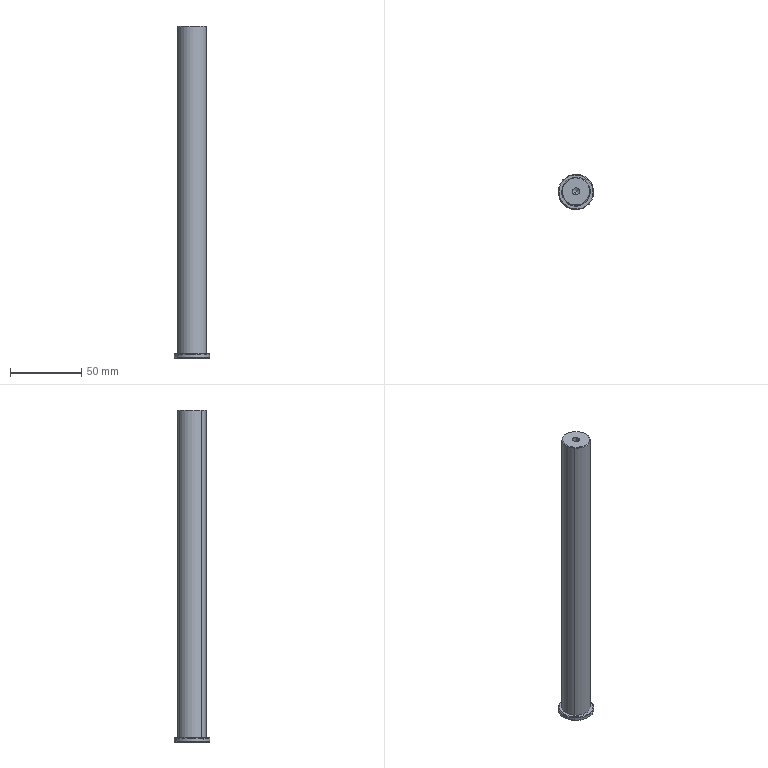Component | SolidWorks | JYTBJ-HeaderPlateRotatingAxis-1 | 1 solid | 17 faces | box 25 x 25 x 233 mm | volume 73359 mm3 | cone 8 | cylinder 6 | plane 3 | commonest cylinder face diameters 5 x2 25 x2 20 x2
build123d program:
from build123d import *

# Parameters (mm, degrees)
SKETCH1_R             = 10
BOSS_EXTRUDE1_DEPTH   = 115
SKETCH2_R             = 12.5
BOSS_EXTRUDE2_DEPTH   = 3
CHAMFER1_SIZE         = 0.5
M6_TAPPED_HOLE1_D     = 5
M6_TAPPED_HOLE1_DEPTH = 17
M6_TAPPED_HOLE1_TIP   = 1.502


with BuildPart() as part:
    # Sketch1 → Boss-Extrude1 (new, symmetric)
    with BuildSketch(Plane.XY):
        Circle(SKETCH1_R)
    extrude(amount=BOSS_EXTRUDE1_DEPTH, both=True)

    # Sketch2 → Boss-Extrude2 (add)
    with BuildSketch(Plane.XY.offset(115)):
        Circle(SKETCH2_R)
    extrude(amount=BOSS_EXTRUDE2_DEPTH)

    # Chamfer1
    chamfer1_edges = [part.edges().sort_by_distance(p)[0] for p in [
        (-10, 0, -115),
        (-12.5, 0, 115),
        (-12.5, 0, 118),
    ]]
    chamfer(chamfer1_edges, length=CHAMFER1_SIZE)

    # M6 Tapped Hole1
    with Locations(Plane(origin=(0, 0, -115), x_dir=(-1, 0, 0), z_dir=(0, 0, -1))):
        with Locations((0, 0)):
            Hole(M6_TAPPED_HOLE1_D / 2, depth=M6_TAPPED_HOLE1_DEPTH)
            with Locations((0, 0, -(M6_TAPPED_HOLE1_DEPTH + M6_TAPPED_HOLE1_TIP / 2))):  # 118° drill point
                Cone(0, M6_TAPPED_HOLE1_D / 2, M6_TAPPED_HOLE1_TIP, mode=Mode.SUBTRACT)


solid = part.part

# Placed as in the assembly
solid = solid.moved(Location((3.373, 96.878, 86), (180, 0, 0)))
STEP:
#1=CARTESIAN_POINT('',(0.05811,3.75,7.244));
#2=VERTEX_POINT('',#1);
#3=CARTESIAN_POINT('',(0.2075,3.878,7.244));
#4=VERTEX_POINT('',#3);
#5=CARTESIAN_POINT('',(0.1328,3.814,7.244));
#6=DIRECTION('',(0.,0.,1.));
#7=DIRECTION('',(0.759,0.6511,0.));
#8=AXIS2_PLACEMENT_3D('',#5,#6,#7);
#9=CIRCLE('',#8,0.09843);
#10=EDGE_CURVE('',#2,#4,#9,.T.);
#11=ORIENTED_EDGE('',*,*,#10,.F.);
#12=CARTESIAN_POINT('',(0.05811,3.75,7.913));
#13=VERTEX_POINT('',#12);
#14=CARTESIAN_POINT('',(0.05811,3.75,7.913));
#15=DIRECTION('',(0.,0.,1.));
#16=VECTOR('',#15,39.37);
#17=LINE('',#14,#16);
#18=EDGE_CURVE('',#2,#13,#17,.T.);
#19=ORIENTED_EDGE('',*,*,#18,.T.);
#20=CARTESIAN_POINT('',(0.2075,3.878,7.913));
#21=VERTEX_POINT('',#20);
#22=CARTESIAN_POINT('',(0.1328,3.814,7.913));
#23=DIRECTION('',(0.,0.,1.));
#24=DIRECTION('',(0.759,0.6511,0.));
#25=AXIS2_PLACEMENT_3D('',#22,#23,#24);
#26=CIRCLE('',#25,0.09843);
#27=EDGE_CURVE('',#13,#21,#26,.T.);
#28=ORIENTED_EDGE('',*,*,#27,.T.);
#29=CARTESIAN_POINT('',(0.2075,3.878,7.913));
#30=DIRECTION('',(0.,0.,1.));
#31=VECTOR('',#30,39.37);
#32=LINE('',#29,#31);
#33=EDGE_CURVE('',#4,#21,#32,.T.);
#34=ORIENTED_EDGE('',*,*,#33,.F.);
#35=EDGE_LOOP('',(#11,#19,#28,#34));
#36=FACE_OUTER_BOUND('',#35,.T.);
#37=CARTESIAN_POINT('',(0.1328,3.814,7.913));
#38=DIRECTION('',(0.,0.,1.));
#39=DIRECTION('',(0.759,0.6511,0.));
#40=AXIS2_PLACEMENT_3D('',#37,#38,#39);
#41=CYLINDRICAL_SURFACE('',#40,0.09843);
#42=ADVANCED_FACE('',(#36),#41,.F.);
#43=CARTESIAN_POINT('',(0.1328,3.814,7.185));
#44=VERTEX_POINT('',#43);
#45=CARTESIAN_POINT('',(0.2075,3.878,7.244));
#46=DIRECTION('',(0.6506,0.5581,0.515));
#47=VECTOR('',#46,39.37);
#48=LINE('',#45,#47);
#49=EDGE_CURVE('',#44,#4,#48,.T.);
#50=ORIENTED_EDGE('',*,*,#49,.F.);
#51=CARTESIAN_POINT('',(0.05811,3.75,7.244));
#52=DIRECTION('',(-0.6506,-0.5581,0.515));
#53=VECTOR('',#52,39.37);
#54=LINE('',#51,#53);
#55=EDGE_CURVE('',#44,#2,#54,.T.);
#56=ORIENTED_EDGE('',*,*,#55,.T.);
#57=ORIENTED_EDGE('',*,*,#10,.T.);
#58=EDGE_LOOP('',(#50,#56,#57));
#59=FACE_OUTER_BOUND('',#58,.T.);
#60=CARTESIAN_POINT('',(0.1328,3.814,7.244));
#61=DIRECTION('',(0.,0.,1.));
#62=DIRECTION('',(0.759,0.6511,0.));
#63=AXIS2_PLACEMENT_3D('',#60,#61,#62);
#64=CONICAL_SURFACE('',#63,0.09843,1.03);
#65=ADVANCED_FACE('',(#59),#64,.F.);
#66=CARTESIAN_POINT('',(0.4167,4.058,7.913));
#67=VERTEX_POINT('',#66);
#68=CARTESIAN_POINT('',(-0.1511,3.571,7.913));
#69=VERTEX_POINT('',#68);
#70=CARTESIAN_POINT('',(0.1328,3.814,7.913));
#71=DIRECTION('',(0.,0.,1.));
#72=DIRECTION('',(-0.759,-0.6511,0.));
#73=AXIS2_PLACEMENT_3D('',#70,#71,#72);
#74=CIRCLE('',#73,0.374);
#75=EDGE_CURVE('',#67,#69,#74,.T.);
#76=ORIENTED_EDGE('',*,*,#75,.F.);
#77=CARTESIAN_POINT('',(0.4316,4.07,7.894));
#78=VERTEX_POINT('',#77);
#79=CARTESIAN_POINT('',(0.4316,4.07,7.894));
#80=DIRECTION('',(0.5367,0.4604,-0.7071));
#81=VECTOR('',#80,39.37);
#82=LINE('',#79,#81);
#83=EDGE_CURVE('',#67,#78,#82,.T.);
#84=ORIENTED_EDGE('',*,*,#83,.T.);
#85=CARTESIAN_POINT('',(-0.166,3.558,7.894));
#86=VERTEX_POINT('',#85);
#87=CARTESIAN_POINT('',(0.1328,3.814,7.894));
#88=DIRECTION('',(0.,0.,-1.));
#89=DIRECTION('',(-0.759,-0.6511,0.));
#90=AXIS2_PLACEMENT_3D('',#87,#88,#89);
#91=CIRCLE('',#90,0.3937);
#92=EDGE_CURVE('',#86,#78,#91,.T.);
#93=ORIENTED_EDGE('',*,*,#92,.F.);
#94=CARTESIAN_POINT('',(-0.166,3.558,7.894));
#95=DIRECTION('',(-0.5367,-0.4604,-0.7071));
#96=VECTOR('',#95,39.37);
#97=LINE('',#94,#96);
#98=EDGE_CURVE('',#69,#86,#97,.T.);
#99=ORIENTED_EDGE('',*,*,#98,.F.);
#100=EDGE_LOOP('',(#76,#84,#93,#99));
#101=FACE_OUTER_BOUND('',#100,.T.);
#102=CARTESIAN_POINT('',(0.1328,3.814,7.894));
#103=DIRECTION('',(0.,0.,-1.));
#104=DIRECTION('',(-0.759,-0.6511,0.));
#105=AXIS2_PLACEMENT_3D('',#102,#103,#104);
#106=CONICAL_SURFACE('',#105,0.3937,0.7854);
#107=ADVANCED_FACE('',(#101),#106,.T.);
#108=CARTESIAN_POINT('',(-0.2258,3.506,-1.26));
#109=VERTEX_POINT('',#108);
#110=CARTESIAN_POINT('',(0.4914,4.122,-1.26));
#111=VERTEX_POINT('',#110);
#112=CARTESIAN_POINT('',(0.1328,3.814,-1.26));
#113=DIRECTION('',(0.,0.,-1.));
#114=DIRECTION('',(-0.759,-0.6511,0.));
#115=AXIS2_PLACEMENT_3D('',#112,#113,#114);
#116=CIRCLE('',#115,0.4724);
#117=EDGE_CURVE('',#109,#111,#116,.T.);
#118=ORIENTED_EDGE('',*,*,#117,.F.);
#119=CARTESIAN_POINT('',(-0.2407,3.494,-1.24));
#120=VERTEX_POINT('',#119);
#121=CARTESIAN_POINT('',(-0.2258,3.506,-1.26));
#122=DIRECTION('',(-0.5367,-0.4604,0.7071));
#123=VECTOR('',#122,39.37);
#124=LINE('',#121,#123);
#125=EDGE_CURVE('',#109,#120,#124,.T.);
#126=ORIENTED_EDGE('',*,*,#125,.T.);
#127=CARTESIAN_POINT('',(0.5063,4.135,-1.24));
#128=VERTEX_POINT('',#127);
#129=CARTESIAN_POINT('',(0.1328,3.814,-1.24));
#130=DIRECTION('',(0.,0.,1.));
#131=DIRECTION('',(-0.759,-0.6511,0.));
#132=AXIS2_PLACEMENT_3D('',#129,#130,#131);
#133=CIRCLE('',#132,0.4921);
#134=EDGE_CURVE('',#128,#120,#133,.T.);
#135=ORIENTED_EDGE('',*,*,#134,.F.);
#136=CARTESIAN_POINT('',(0.4914,4.122,-1.26));
#137=DIRECTION('',(0.5367,0.4604,0.7071));
#138=VECTOR('',#137,39.37);
#139=LINE('',#136,#138);
#140=EDGE_CURVE('',#111,#128,#139,.T.);
#141=ORIENTED_EDGE('',*,*,#140,.F.);
#142=EDGE_LOOP('',(#118,#126,#135,#141));
#143=FACE_OUTER_BOUND('',#142,.T.);
#144=CARTESIAN_POINT('',(0.1328,3.814,-1.26));
#145=DIRECTION('',(0.,0.,1.));
#146=DIRECTION('',(0.759,0.6511,0.));
#147=AXIS2_PLACEMENT_3D('',#144,#145,#146);
#148=CONICAL_SURFACE('',#147,0.4724,0.7854);
#149=ADVANCED_FACE('',(#143),#148,.T.);
#150=CARTESIAN_POINT('',(0.4914,4.122,-1.142));
#151=VERTEX_POINT('',#150);
#152=CARTESIAN_POINT('',(-0.2258,3.506,-1.142));
#153=VERTEX_POINT('',#152);
#154=CARTESIAN_POINT('',(0.1328,3.814,-1.142));
#155=DIRECTION('',(0.,0.,1.));
#156=DIRECTION('',(-0.759,-0.6511,0.));
#157=AXIS2_PLACEMENT_3D('',#154,#155,#156);
#158=CIRCLE('',#157,0.4724);
#159=EDGE_CURVE('',#151,#153,#158,.T.);
#160=ORIENTED_EDGE('',*,*,#159,.F.);
#161=CARTESIAN_POINT('',(0.5063,4.135,-1.161));
#162=VERTEX_POINT('',#161);
#163=CARTESIAN_POINT('',(0.5063,4.135,-1.161));
#164=DIRECTION('',(0.5367,0.4604,-0.7071));
#165=VECTOR('',#164,39.37);
#166=LINE('',#163,#165);
#167=EDGE_CURVE('',#151,#162,#166,.T.);
#168=ORIENTED_EDGE('',*,*,#167,.T.);
#169=CARTESIAN_POINT('',(-0.2407,3.494,-1.161));
#170=VERTEX_POINT('',#169);
#171=CARTESIAN_POINT('',(0.1328,3.814,-1.161));
#172=DIRECTION('',(0.,0.,-1.));
#173=DIRECTION('',(-0.759,-0.6511,0.));
#174=AXIS2_PLACEMENT_3D('',#171,#172,#173);
#175=CIRCLE('',#174,0.4921);
#176=EDGE_CURVE('',#170,#162,#175,.T.);
#177=ORIENTED_EDGE('',*,*,#176,.F.);
#178=CARTESIAN_POINT('',(-0.2407,3.494,-1.161));
#179=DIRECTION('',(-0.5367,-0.4604,-0.7071));
#180=VECTOR('',#179,39.37);
#181=LINE('',#178,#180);
#182=EDGE_CURVE('',#153,#170,#181,.T.);
#183=ORIENTED_EDGE('',*,*,#182,.F.);
#184=EDGE_LOOP('',(#160,#168,#177,#183));
#185=FACE_OUTER_BOUND('',#184,.T.);
#186=CARTESIAN_POINT('',(0.1328,3.814,-1.161));
#187=DIRECTION('',(0.,0.,-1.));
#188=DIRECTION('',(-0.759,-0.6511,0.));
#189=AXIS2_PLACEMENT_3D('',#186,#187,#188);
#190=CONICAL_SURFACE('',#189,0.4921,0.7854);
#191=ADVANCED_FACE('',(#185),#190,.T.);
#192=ORIENTED_EDGE('',*,*,#134,.T.);
#193=CARTESIAN_POINT('',(-0.2407,3.494,-1.26));
#194=DIRECTION('',(0.,0.,1.));
#195=VECTOR('',#194,39.37);
#196=LINE('',#193,#195);
#197=EDGE_CURVE('',#120,#170,#196,.T.);
#198=ORIENTED_EDGE('',*,*,#197,.T.);
#199=ORIENTED_EDGE('',*,*,#176,.T.);
#200=CARTESIAN_POINT('',(0.5063,4.135,-1.26));
#201=DIRECTION('',(0.,0.,1.));
#202=VECTOR('',#201,39.37);
#203=LINE('',#200,#202);
#204=EDGE_CURVE('',#128,#162,#203,.T.);
#205=ORIENTED_EDGE('',*,*,#204,.F.);
#206=EDGE_LOOP('',(#192,#198,#199,#205));
#207=FACE_OUTER_BOUND('',#206,.T.);
#208=CARTESIAN_POINT('',(0.1328,3.814,-1.26));
#209=DIRECTION('',(0.,0.,1.));
#210=DIRECTION('',(0.759,0.6511,0.));
#211=AXIS2_PLACEMENT_3D('',#208,#209,#210);
#212=CYLINDRICAL_SURFACE('',#211,0.4921);
#213=ADVANCED_FACE('',(#207),#212,.T.);
#214=CARTESIAN_POINT('',(-0.166,3.558,-1.142));
#215=VERTEX_POINT('',#214);
#216=CARTESIAN_POINT('',(0.4316,4.07,-1.142));
#217=VERTEX_POINT('',#216);
#218=CARTESIAN_POINT('',(0.1328,3.814,-1.142));
#219=DIRECTION('',(0.,0.,-1.));
#220=DIRECTION('',(-0.759,-0.6511,0.));
#221=AXIS2_PLACEMENT_3D('',#218,#219,#220);
#222=CIRCLE('',#221,0.3937);
#223=EDGE_CURVE('',#215,#217,#222,.T.);
#224=ORIENTED_EDGE('',*,*,#223,.F.);
#225=CARTESIAN_POINT('',(-0.166,3.558,-1.142));
#226=DIRECTION('',(0.,0.,1.));
#227=VECTOR('',#226,39.37);
#228=LINE('',#225,#227);
#229=EDGE_CURVE('',#215,#86,#228,.T.);
#230=ORIENTED_EDGE('',*,*,#229,.T.);
#231=ORIENTED_EDGE('',*,*,#92,.T.);
#232=CARTESIAN_POINT('',(0.4316,4.07,-1.142));
#233=DIRECTION('',(0.,0.,1.));
#234=VECTOR('',#233,39.37);
#235=LINE('',#232,#234);
#236=EDGE_CURVE('',#217,#78,#235,.T.);
#237=ORIENTED_EDGE('',*,*,#236,.F.);
#238=EDGE_LOOP('',(#224,#230,#231,#237));
#239=FACE_OUTER_BOUND('',#238,.T.);
#240=CARTESIAN_POINT('',(0.1328,3.814,-1.142));
#241=DIRECTION('',(0.,0.,1.));
#242=DIRECTION('',(0.759,0.6511,0.));
#243=AXIS2_PLACEMENT_3D('',#240,#241,#242);
#244=CYLINDRICAL_SURFACE('',#243,0.3937);
#245=ADVANCED_FACE('',(#239),#244,.T.);
#246=ORIENTED_EDGE('',*,*,#229,.F.);
#247=CARTESIAN_POINT('',(0.1328,3.814,-1.142));
#248=DIRECTION('',(0.,0.,-1.));
#249=DIRECTION('',(-0.759,-0.6511,0.));
#250=AXIS2_PLACEMENT_3D('',#247,#248,#249);
#251=CIRCLE('',#250,0.3937);
#252=EDGE_CURVE('',#217,#215,#251,.T.);
#253=ORIENTED_EDGE('',*,*,#252,.F.);
#254=ORIENTED_EDGE('',*,*,#236,.T.);
#255=CARTESIAN_POINT('',(0.1328,3.814,7.894));
#256=DIRECTION('',(0.,0.,-1.));
#257=DIRECTION('',(-0.759,-0.6511,0.));
#258=AXIS2_PLACEMENT_3D('',#255,#256,#257);
#259=CIRCLE('',#258,0.3937);
#260=EDGE_CURVE('',#78,#86,#259,.T.);
#261=ORIENTED_EDGE('',*,*,#260,.T.);
#262=EDGE_LOOP('',(#246,#253,#254,#261));
#263=FACE_OUTER_BOUND('',#262,.T.);
#264=CARTESIAN_POINT('',(0.1328,3.814,-1.142));
#265=DIRECTION('',(0.,0.,1.));
#266=DIRECTION('',(0.759,0.6511,0.));
#267=AXIS2_PLACEMENT_3D('',#264,#265,#266);
#268=CYLINDRICAL_SURFACE('',#267,0.3937);
#269=ADVANCED_FACE('',(#263),#268,.T.);
#270=CARTESIAN_POINT('',(0.1328,3.814,7.913));
#271=DIRECTION('',(0.,0.,1.));
#272=DIRECTION('',(0.759,0.6511,0.));
#273=AXIS2_PLACEMENT_3D('',#270,#271,#272);
#274=CIRCLE('',#273,0.09843);
#275=EDGE_CURVE('',#21,#13,#274,.T.);
#276=ORIENTED_EDGE('',*,*,#275,.F.);
#277=ORIENTED_EDGE('',*,*,#27,.F.);
#278=EDGE_LOOP('',(#276,#277));
#279=FACE_BOUND('',#278,.T.);
#280=CARTESIAN_POINT('',(0.1328,3.814,7.913));
#281=DIRECTION('',(0.,0.,1.));
#282=DIRECTION('',(-0.759,-0.6511,0.));
#283=AXIS2_PLACEMENT_3D('',#280,#281,#282);
#284=CIRCLE('',#283,0.374);
#285=EDGE_CURVE('',#69,#67,#284,.T.);
#286=ORIENTED_EDGE('',*,*,#285,.T.);
#287=ORIENTED_EDGE('',*,*,#75,.T.);
#288=EDGE_LOOP('',(#286,#287));
#289=FACE_OUTER_BOUND('',#288,.T.);
#290=CARTESIAN_POINT('',(0.1328,3.814,7.913));
#291=DIRECTION('',(0.,0.,-1.));
#292=DIRECTION('',(-0.759,-0.6511,0.));
#293=AXIS2_PLACEMENT_3D('',#290,#291,#292);
#294=PLANE('',#293);
#295=ADVANCED_FACE('',(#279,#289),#294,.F.);
#296=CARTESIAN_POINT('',(0.1328,3.814,-1.142));
#297=DIRECTION('',(0.,0.,1.));
#298=DIRECTION('',(-0.759,-0.6511,0.));
#299=AXIS2_PLACEMENT_3D('',#296,#297,#298);
#300=CIRCLE('',#299,0.4724);
#301=EDGE_CURVE('',#153,#151,#300,.T.);
#302=ORIENTED_EDGE('',*,*,#301,.T.);
#303=ORIENTED_EDGE('',*,*,#159,.T.);
#304=EDGE_LOOP('',(#302,#303));
#305=FACE_OUTER_BOUND('',#304,.T.);
#306=ORIENTED_EDGE('',*,*,#252,.T.);
#307=ORIENTED_EDGE('',*,*,#223,.T.);
#308=EDGE_LOOP('',(#306,#307));
#309=FACE_BOUND('',#308,.T.);
#310=CARTESIAN_POINT('',(0.1328,3.814,-1.142));
#311=DIRECTION('',(0.,0.,-1.));
#312=DIRECTION('',(-0.759,-0.6511,0.));
#313=AXIS2_PLACEMENT_3D('',#310,#311,#312);
#314=PLANE('',#313);
#315=ADVANCED_FACE('',(#305,#309),#314,.F.);
#316=ORIENTED_EDGE('',*,*,#197,.F.);
#317=CARTESIAN_POINT('',(0.1328,3.814,-1.24));
#318=DIRECTION('',(0.,0.,1.));
#319=DIRECTION('',(-0.759,-0.6511,0.));
#320=AXIS2_PLACEMENT_3D('',#317,#318,#319);
#321=CIRCLE('',#320,0.4921);
#322=EDGE_CURVE('',#120,#128,#321,.T.);
#323=ORIENTED_EDGE('',*,*,#322,.T.);
#324=ORIENTED_EDGE('',*,*,#204,.T.);
#325=CARTESIAN_POINT('',(0.1328,3.814,-1.161));
#326=DIRECTION('',(0.,0.,-1.));
#327=DIRECTION('',(-0.759,-0.6511,0.));
#328=AXIS2_PLACEMENT_3D('',#325,#326,#327);
#329=CIRCLE('',#328,0.4921);
#330=EDGE_CURVE('',#162,#170,#329,.T.);
#331=ORIENTED_EDGE('',*,*,#330,.T.);
#332=EDGE_LOOP('',(#316,#323,#324,#331));
#333=FACE_OUTER_BOUND('',#332,.T.);
#334=CARTESIAN_POINT('',(0.1328,3.814,-1.26));
#335=DIRECTION('',(0.,0.,1.));
#336=DIRECTION('',(0.759,0.6511,0.));
#337=AXIS2_PLACEMENT_3D('',#334,#335,#336);
#338=CYLINDRICAL_SURFACE('',#337,0.4921);
#339=ADVANCED_FACE('',(#333),#338,.T.);
#340=CARTESIAN_POINT('',(0.1328,3.814,-1.26));
#341=DIRECTION('',(0.,0.,-1.));
#342=DIRECTION('',(-0.759,-0.6511,0.));
#343=AXIS2_PLACEMENT_3D('',#340,#341,#342);
#344=CIRCLE('',#343,0.4724);
#345=EDGE_CURVE('',#111,#109,#344,.T.);
#346=ORIENTED_EDGE('',*,*,#345,.T.);
#347=ORIENTED_EDGE('',*,*,#117,.T.);
#348=EDGE_LOOP('',(#346,#347));
#349=FACE_OUTER_BOUND('',#348,.T.);
#350=CARTESIAN_POINT('',(0.1328,3.814,-1.26));
#351=DIRECTION('',(0.,0.,-1.));
#352=DIRECTION('',(-0.759,-0.6511,0.));
#353=AXIS2_PLACEMENT_3D('',#350,#351,#352);
#354=PLANE('',#353);
#355=ADVANCED_FACE('',(#349),#354,.T.);
#356=ORIENTED_EDGE('',*,*,#167,.F.);
#357=ORIENTED_EDGE('',*,*,#301,.F.);
#358=ORIENTED_EDGE('',*,*,#182,.T.);
#359=ORIENTED_EDGE('',*,*,#330,.F.);
#360=EDGE_LOOP('',(#356,#357,#358,#359));
#361=FACE_OUTER_BOUND('',#360,.T.);
#362=CARTESIAN_POINT('',(0.1328,3.814,-1.161));
#363=DIRECTION('',(0.,0.,-1.));
#364=DIRECTION('',(-0.759,-0.6511,0.));
#365=AXIS2_PLACEMENT_3D('',#362,#363,#364);
#366=CONICAL_SURFACE('',#365,0.4921,0.7854);
#367=ADVANCED_FACE('',(#361),#366,.T.);
#368=ORIENTED_EDGE('',*,*,#125,.F.);
#369=ORIENTED_EDGE('',*,*,#345,.F.);
#370=ORIENTED_EDGE('',*,*,#140,.T.);
#371=ORIENTED_EDGE('',*,*,#322,.F.);
#372=EDGE_LOOP('',(#368,#369,#370,#371));
#373=FACE_OUTER_BOUND('',#372,.T.);
#374=CARTESIAN_POINT('',(0.1328,3.814,-1.26));
#375=DIRECTION('',(0.,0.,1.));
#376=DIRECTION('',(0.759,0.6511,0.));
#377=AXIS2_PLACEMENT_3D('',#374,#375,#376);
#378=CONICAL_SURFACE('',#377,0.4724,0.7854);
#379=ADVANCED_FACE('',(#373),#378,.T.);
#380=ORIENTED_EDGE('',*,*,#83,.F.);
#381=ORIENTED_EDGE('',*,*,#285,.F.);
#382=ORIENTED_EDGE('',*,*,#98,.T.);
#383=ORIENTED_EDGE('',*,*,#260,.F.);
#384=EDGE_LOOP('',(#380,#381,#382,#383));
#385=FACE_OUTER_BOUND('',#384,.T.);
#386=CARTESIAN_POINT('',(0.1328,3.814,7.894));
#387=DIRECTION('',(0.,0.,-1.));
#388=DIRECTION('',(-0.759,-0.6511,0.));
#389=AXIS2_PLACEMENT_3D('',#386,#387,#388);
#390=CONICAL_SURFACE('',#389,0.3937,0.7854);
#391=ADVANCED_FACE('',(#385),#390,.T.);
#392=ORIENTED_EDGE('',*,*,#55,.F.);
#393=ORIENTED_EDGE('',*,*,#49,.T.);
#394=CARTESIAN_POINT('',(0.1328,3.814,7.244));
#395=DIRECTION('',(0.,0.,1.));
#396=DIRECTION('',(0.759,0.6511,0.));
#397=AXIS2_PLACEMENT_3D('',#394,#395,#396);
#398=CIRCLE('',#397,0.09843);
#399=EDGE_CURVE('',#4,#2,#398,.T.);
#400=ORIENTED_EDGE('',*,*,#399,.T.);
#401=EDGE_LOOP('',(#392,#393,#400));
#402=FACE_OUTER_BOUND('',#401,.T.);
#403=CARTESIAN_POINT('',(0.1328,3.814,7.244));
#404=DIRECTION('',(0.,0.,1.));
#405=DIRECTION('',(0.759,0.6511,0.));
#406=AXIS2_PLACEMENT_3D('',#403,#404,#405);
#407=CONICAL_SURFACE('',#406,0.09843,1.03);
#408=ADVANCED_FACE('',(#402),#407,.F.);
#409=ORIENTED_EDGE('',*,*,#18,.F.);
#410=ORIENTED_EDGE('',*,*,#399,.F.);
#411=ORIENTED_EDGE('',*,*,#33,.T.);
#412=ORIENTED_EDGE('',*,*,#275,.T.);
#413=EDGE_LOOP('',(#409,#410,#411,#412));
#414=FACE_OUTER_BOUND('',#413,.T.);
#415=CARTESIAN_POINT('',(0.1328,3.814,7.913));
#416=DIRECTION('',(0.,0.,1.));
#417=DIRECTION('',(0.759,0.6511,0.));
#418=AXIS2_PLACEMENT_3D('',#415,#416,#417);
#419=CYLINDRICAL_SURFACE('',#418,0.09843);
#420=ADVANCED_FACE('',(#414),#419,.F.);
#421=CLOSED_SHELL('',(#42,#65,#107,#149,#191,#213,#245,#269,#295,#315,#339,#355,#367,#379,#391,#408,#420));
#422=MANIFOLD_SOLID_BREP('',#421);
#423=CARTESIAN_POINT('',(0.,0.,0.));
#424=DIRECTION('',(0.,0.,1.));
#425=DIRECTION('',(1.,0.,0.));
#426=AXIS2_PLACEMENT_3D('',#423,#424,#425);
#427=(LENGTH_UNIT()NAMED_UNIT(*)SI_UNIT($,.METRE.));
#428=LENGTH_MEASURE_WITH_UNIT(LENGTH_MEASURE(0.0254),#427);
#429=DIMENSIONAL_EXPONENTS(1.,0.,0.,0.,0.,0.,0.);
#430=(CONVERSION_BASED_UNIT('',#428)LENGTH_UNIT()NAMED_UNIT(#429));
#431=UNCERTAINTY_MEASURE_WITH_UNIT(LENGTH_MEASURE(0.00001),#430,'','');
#432=(NAMED_UNIT(*)PLANE_ANGLE_UNIT()SI_UNIT($,.RADIAN.));
#433=(NAMED_UNIT(*)SI_UNIT($,.STERADIAN.)SOLID_ANGLE_UNIT());
#434=(GEOMETRIC_REPRESENTATION_CONTEXT(3)GLOBAL_UNCERTAINTY_ASSIGNED_CONTEXT((#431))GLOBAL_UNIT_ASSIGNED_CONTEXT((#430,#432,#433))REPRESENTATION_CONTEXT('',''));
#435=ADVANCED_BREP_SHAPE_REPRESENTATION('',(#422,#426),#434);
#436=COLOUR_RGB('',0.7922,0.8196,0.9333);
#437=FILL_AREA_STYLE_COLOUR('',#436);
#438=FILL_AREA_STYLE('',(#437));
#439=SURFACE_STYLE_FILL_AREA(#438);
#440=SURFACE_SIDE_STYLE('',(#439));
#441=SURFACE_STYLE_USAGE(.BOTH.,#440);
#442=PRESENTATION_STYLE_ASSIGNMENT((#441));
#443=STYLED_ITEM('',(#442),#422);
#444=PRESENTATION_LAYER_ASSIGNMENT('','',(#443));
#445=(LENGTH_UNIT()NAMED_UNIT(*)SI_UNIT($,.METRE.));
#446=LENGTH_MEASURE_WITH_UNIT(LENGTH_MEASURE(0.0254),#445);
#447=DIMENSIONAL_EXPONENTS(1.,0.,0.,0.,0.,0.,0.);
#448=(CONVERSION_BASED_UNIT('',#446)LENGTH_UNIT()NAMED_UNIT(#447));
#449=UNCERTAINTY_MEASURE_WITH_UNIT(LENGTH_MEASURE(0.00001),#448,'','');
#450=(NAMED_UNIT(*)PLANE_ANGLE_UNIT()SI_UNIT($,.RADIAN.));
#451=(NAMED_UNIT(*)SI_UNIT($,.STERADIAN.)SOLID_ANGLE_UNIT());
#452=(GEOMETRIC_REPRESENTATION_CONTEXT(3)GLOBAL_UNCERTAINTY_ASSIGNED_CONTEXT((#449))GLOBAL_UNIT_ASSIGNED_CONTEXT((#448,#450,#451))REPRESENTATION_CONTEXT('',''));
#453=MECHANICAL_DESIGN_GEOMETRIC_PRESENTATION_REPRESENTATION('',(#443),#452);